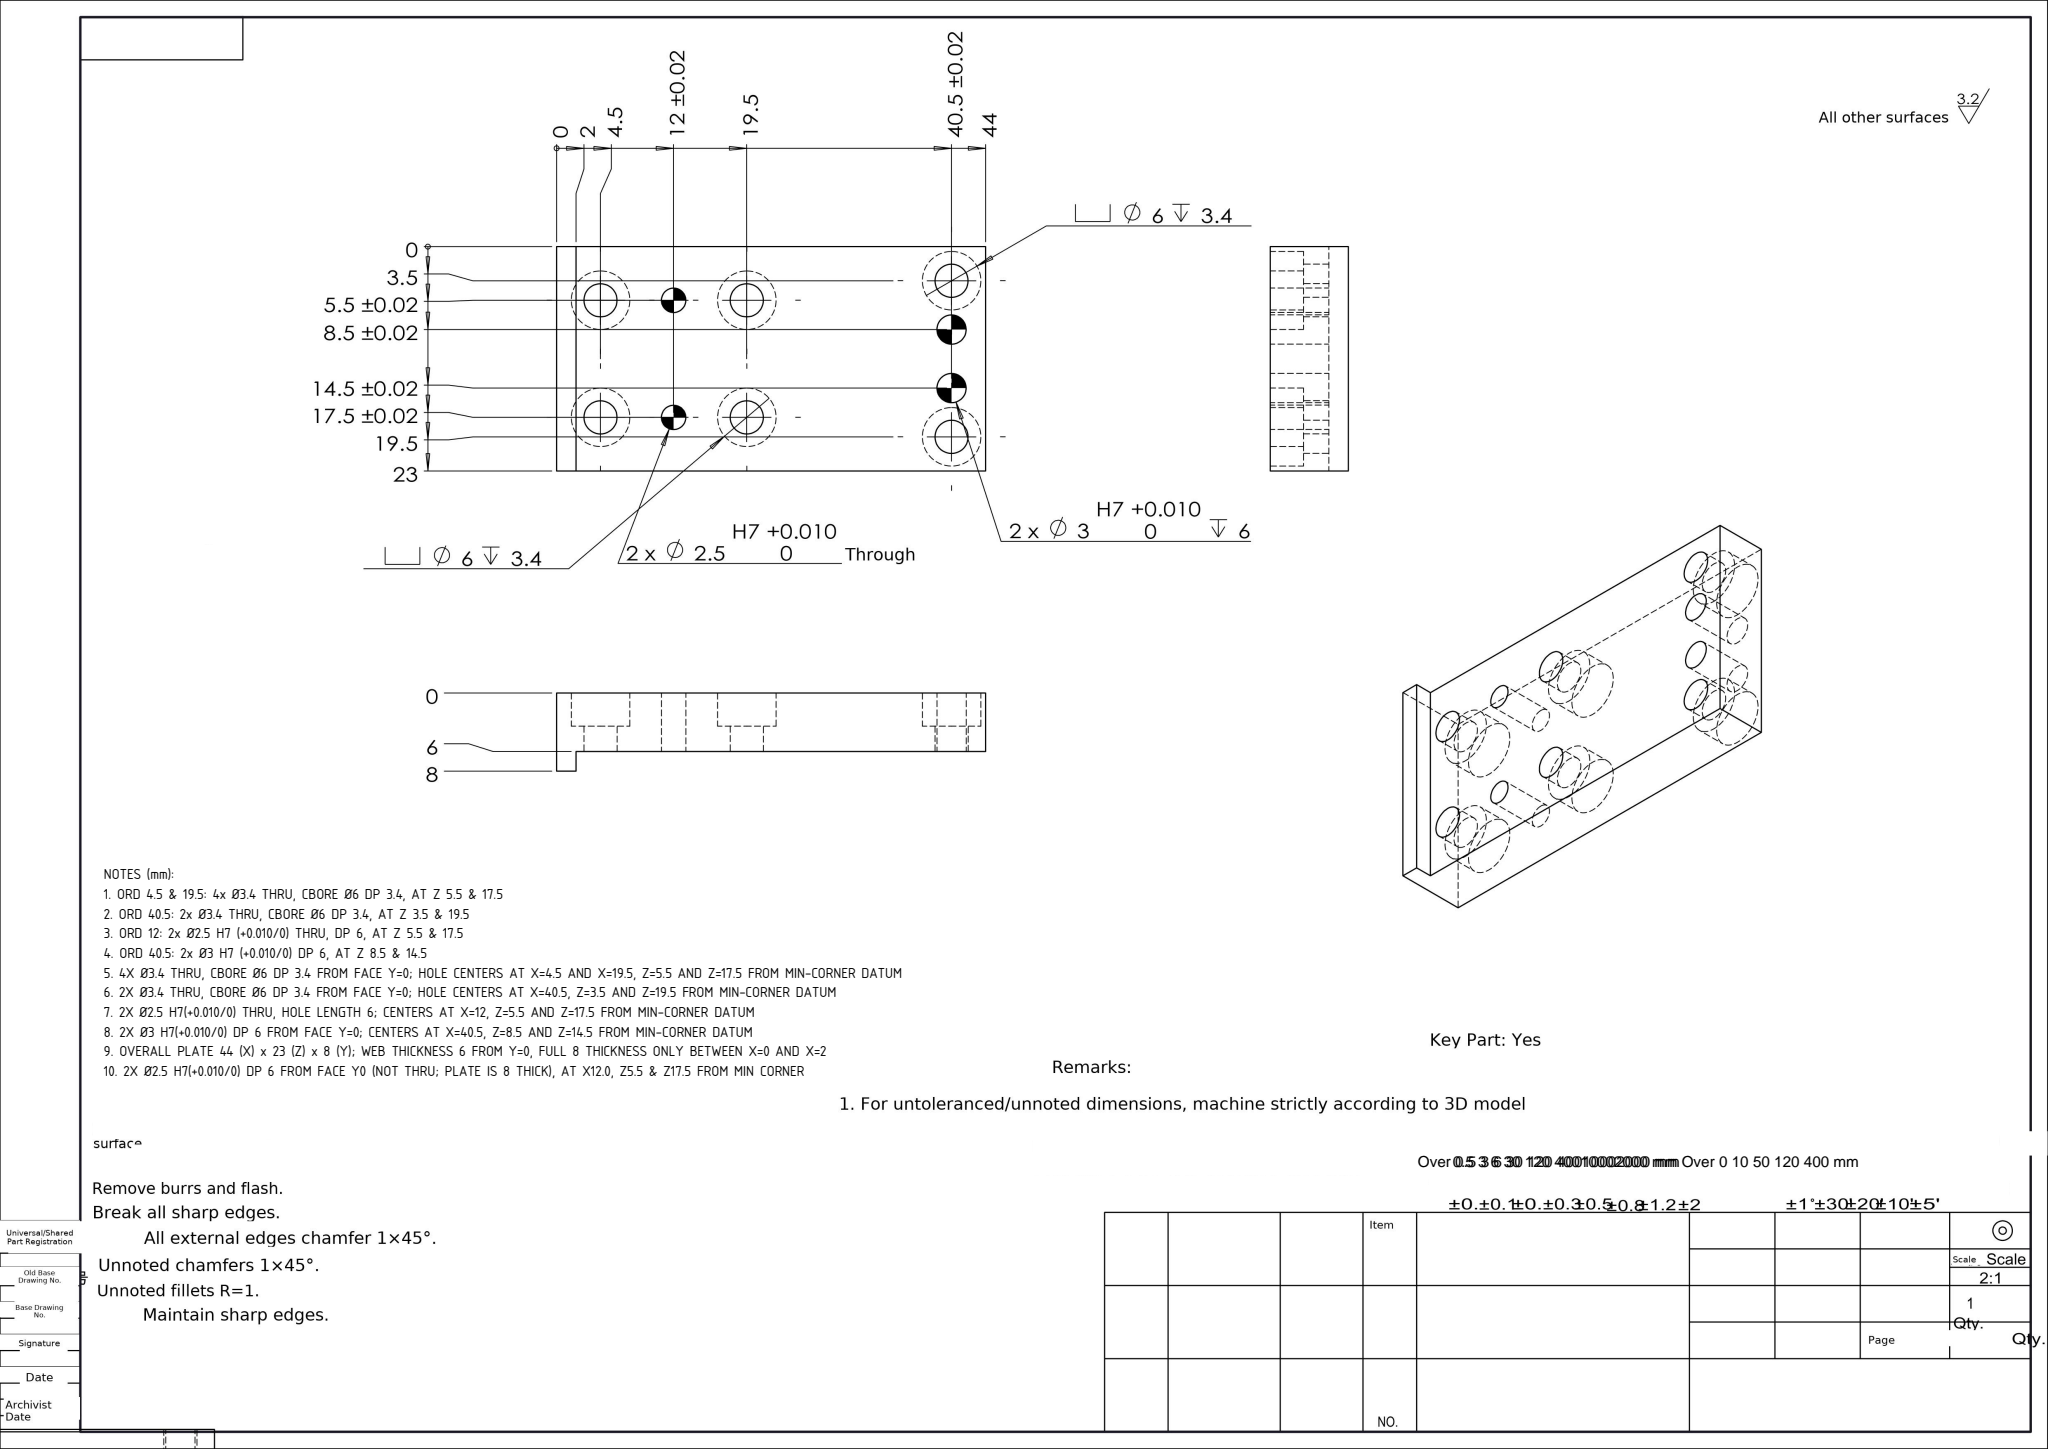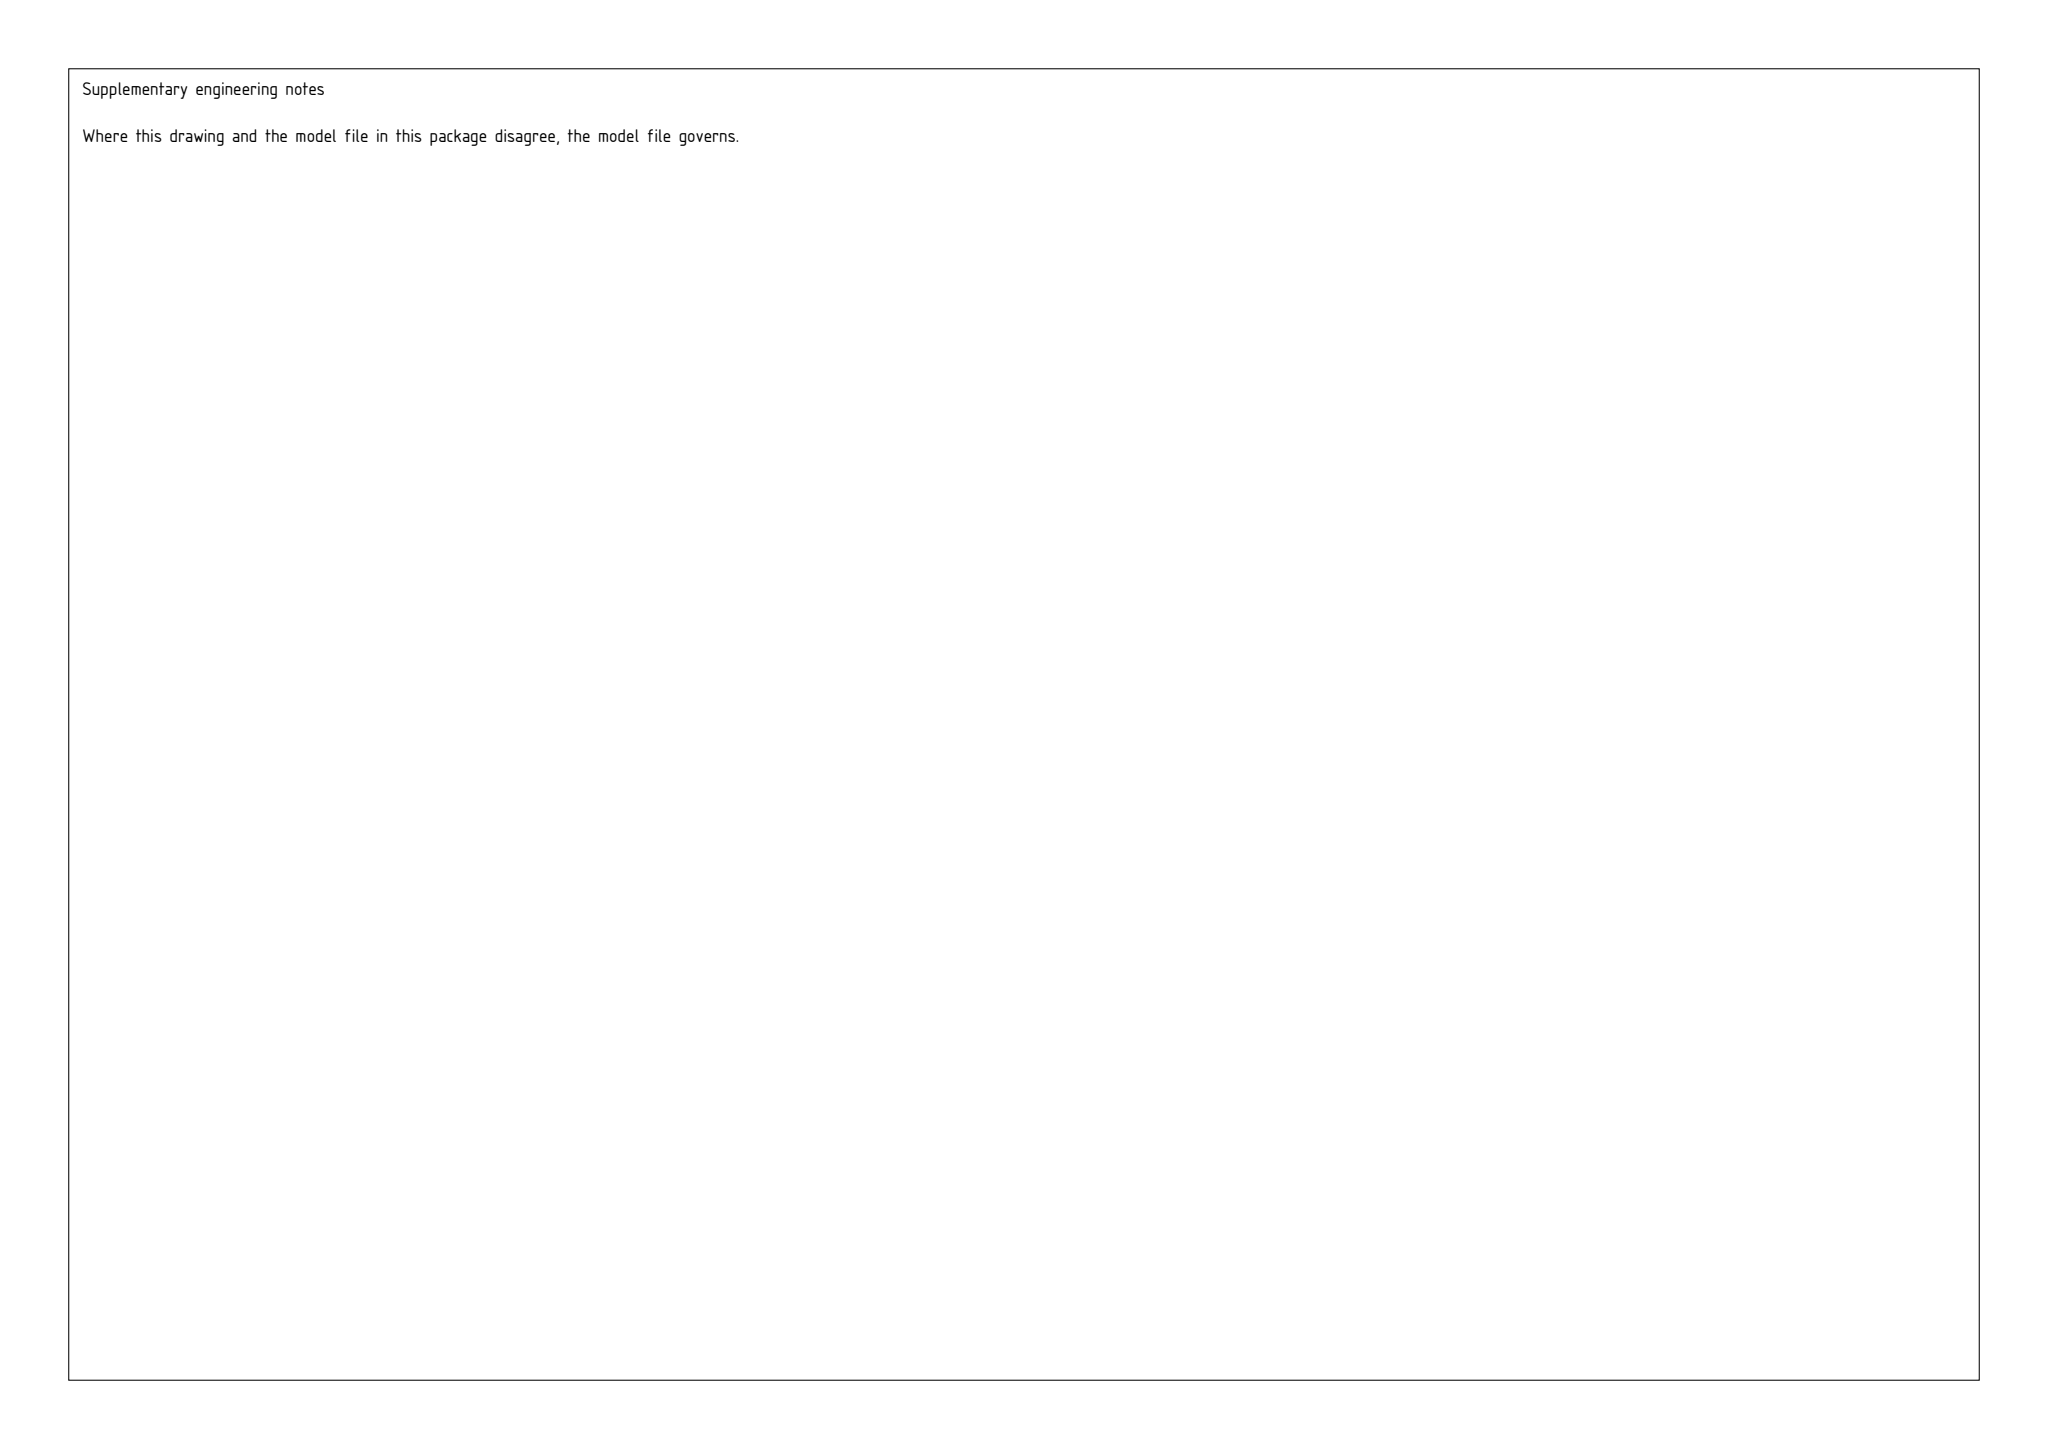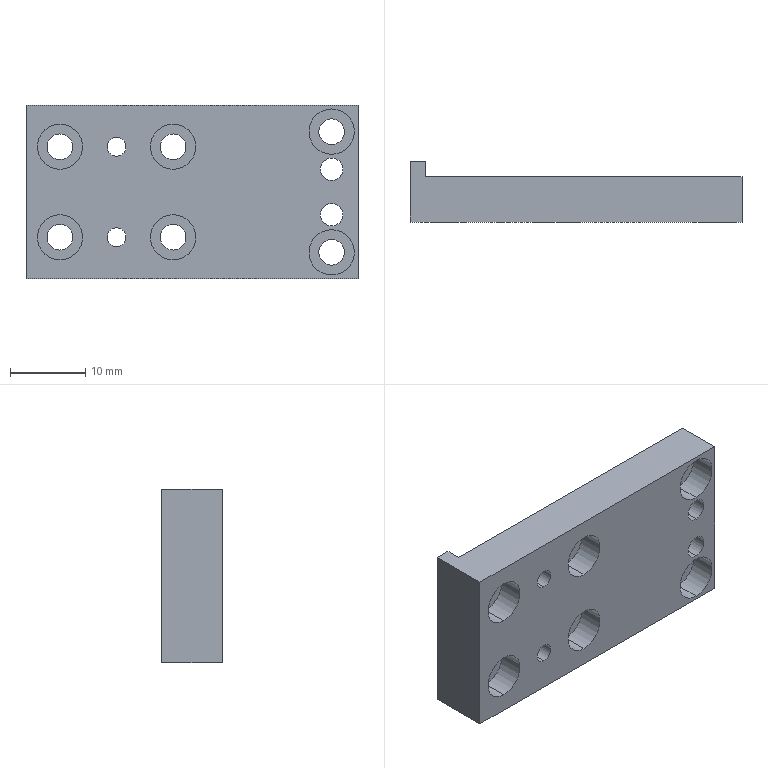Part | SolidWorks | mm | 1 solid | 46 faces | box 44 x 8 x 23 mm | volume 5302 mm3 | cylinder 32 | plane 14 | commonest cylinder face diameters 6 x12 3.4 x12 3 x4 2.5 x4
Drawing notes:
ORD 4.5 & 19.5: 4x Ø3.4 THRU, CBORE Ø6 DP 3.4, AT Z 5.5 & 17.5 | from the solid: Ø3.4 axis y at x=4.5/19.5, z=5.5/17.5, len 2.6; Ø6 cbore len 3.4 same axes
ORD 40.5: 2x Ø3.4 THRU, CBORE Ø6 DP 3.4, AT Z 3.5 & 19.5 | from the solid: Ø3.4 axis y at x=40.5, z=3.5/19.5, len 2.6; Ø6 cbore len 3.4 same axes
ORD 12: 2x Ø2.5 H7 (+0.010/0) THRU, DP 6, AT Z 5.5 & 17.5 | from the solid: Ø2.5 axis y, x=12.0, z=5.5 and 17.5, length 6.0 = wall thk
ORD 40.5: 2x Ø3 H7 (+0.010/0) DP 6, AT Z 8.5 & 14.5 | from the solid: Ø3.0 axis y, x=40.5, z=8.5 and 14.5, length 6.0
4X Ø3.4 THRU, CBORE Ø6 DP 3.4 FROM FACE Y=0; HOLE CENTERS AT X=4.5 AND X=19.5, Z=5.5 AND Z=17.5 FROM MIN-CORNER DATUM | from the solid: cylinders [3.4,y,(4.5/19.5, z 5.5/17.5), len 2.6] and [6.0,y,(4.5/19.5, z 5.5/17.5), len 3.4]
2X Ø3.4 THRU, CBORE Ø6 DP 3.4 FROM FACE Y=0; HOLE CENTERS AT X=40.5, Z=3.5 AND Z=19.5 FROM MIN-CORNER DATUM | from the solid: cylinders [3.4,y,(40.5, z 3.5/19.5), len 2.6] and [6.0,y,(40.5, z 3.5/19.5), len 3.4]
2X Ø2.5 H7(+0.010/0) THRU, HOLE LENGTH 6; CENTERS AT X=12, Z=5.5 AND Z=17.5 FROM MIN-CORNER DATUM | from the solid: cylinders [2.5,y,(12.0, z 5.5/17.5), len 6.0]
2X Ø3 H7(+0.010/0) DP 6 FROM FACE Y=0; CENTERS AT X=40.5, Z=8.5 AND Z=14.5 FROM MIN-CORNER DATUM | from the solid: cylinders [3.0,y,(40.5, z 8.5/14.5), len 6.0]
OVERALL PLATE 44 (X) x 23 (Z) x 8 (Y); WEB THICKNESS 6 FROM Y=0, FULL 8 THICKNESS ONLY BETWEEN X=0 AND X=2 | from the solid: bbox_xyz [44,8,23]; axis_planes x=0, x=2, x=44, y=0, y=6, y=8, z=0, z=23
2X Ø2.5 H7(+0.010/0) DP 6 FROM FACE Y0 (NOT THRU; PLATE IS 8 THICK), AT X12.0, Z5.5 & Z17.5 FROM MIN CORNER | from the solid: cylinders dia 2.5, axis y, pos [12.0,null,5.5] and [12.0,null,17.5], length 6.0; bbox_xyz y=8.0
build123d program:
from build123d import *

# Parameters (mm, degrees)
SKETCH1_W                                         = 42
SKETCH1_H                                         = 6
BOSS_EXTRUDE1_DEPTH                               = 23
SKETCH7_W                                         = 23
SKETCH7_H                                         = 8
BOSS_EXTRUDE2_DEPTH                               = 2
HOLE_SIZE_ACCORDING_TO_HEXAGON_SOCKET_D           = 3.4
HOLE_SIZE_ACCORDING_TO_HEXAGON_SOCKET_CBORE_D     = 6
HOLE_SIZE_ACCORDING_TO_HEXAGON_SOCKET_CBORE_DEPTH = 3.4
SIZE_MM_DOWEL_PIN_HOLE_1_D                        = 2.5
HOLE_SIZE_ACCORDING_TO_HEXAGON_SO_2_D             = 3.4
HOLE_SIZE_ACCORDING_TO_HEXAGON_SO_2_CBORE_D       = 6
HOLE_SIZE_ACCORDING_TO_HEXAGON_SO_2_CBORE_DEPTH   = 3.4
SIZE_MM_DOWEL_PIN_HOLE_3_D                        = 3


with BuildPart() as part:
    # Sketch1 → Boss-Extrude1 (new body)
    with BuildSketch(Plane.XY):
        Rectangle(SKETCH1_W, SKETCH1_H)
    extrude(amount=BOSS_EXTRUDE1_DEPTH)

    # Sketch7 → Boss-Extrude2 (add)
    with BuildSketch(Plane.ZY.offset(21)):
        with Locations((11.5, 1)):
            Rectangle(SKETCH7_W, SKETCH7_H)
    extrude(amount=BOSS_EXTRUDE2_DEPTH)

    # Hole Size _ according to_ Hexagon Socket (through all)
    with Locations(Plane(origin=(0, -3, 0), x_dir=(-1, 0, 0), z_dir=(0, -1, 0))):
        with Locations((3.5, -5.5), (18.5, -5.5), (18.5, -17.5), (3.5, -17.5)):
            CounterBoreHole(HOLE_SIZE_ACCORDING_TO_HEXAGON_SOCKET_D / 2, HOLE_SIZE_ACCORDING_TO_HEXAGON_SOCKET_CBORE_D / 2, HOLE_SIZE_ACCORDING_TO_HEXAGON_SOCKET_CBORE_DEPTH)

    # Size mm Dowel Pin Hole 1 (through all)
    with Locations(Plane(origin=(0, -3, 0), x_dir=(-1, 0, 0), z_dir=(0, -1, 0))):
        with Locations((11, -17.5), (11, -5.5)):
            Hole(SIZE_MM_DOWEL_PIN_HOLE_1_D / 2)

    # Hole Size _ according to_ Hexagon So 2 (through all)
    with Locations(Plane(origin=(0, -3, 0), x_dir=(-1, 0, 0), z_dir=(0, -1, 0))):
        with Locations((-17.5, -3.5), (-17.5, -19.5)):
            CounterBoreHole(HOLE_SIZE_ACCORDING_TO_HEXAGON_SO_2_D / 2, HOLE_SIZE_ACCORDING_TO_HEXAGON_SO_2_CBORE_D / 2, HOLE_SIZE_ACCORDING_TO_HEXAGON_SO_2_CBORE_DEPTH)

    # Size mm Dowel Pin Hole 3 (through all)
    with Locations(Plane(origin=(0, -3, 0), x_dir=(-1, 0, 0), z_dir=(0, -1, 0))):
        with Locations((-17.5, -8.5), (-17.5, -14.5)):
            Hole(SIZE_MM_DOWEL_PIN_HOLE_3_D / 2)


solid = part.part